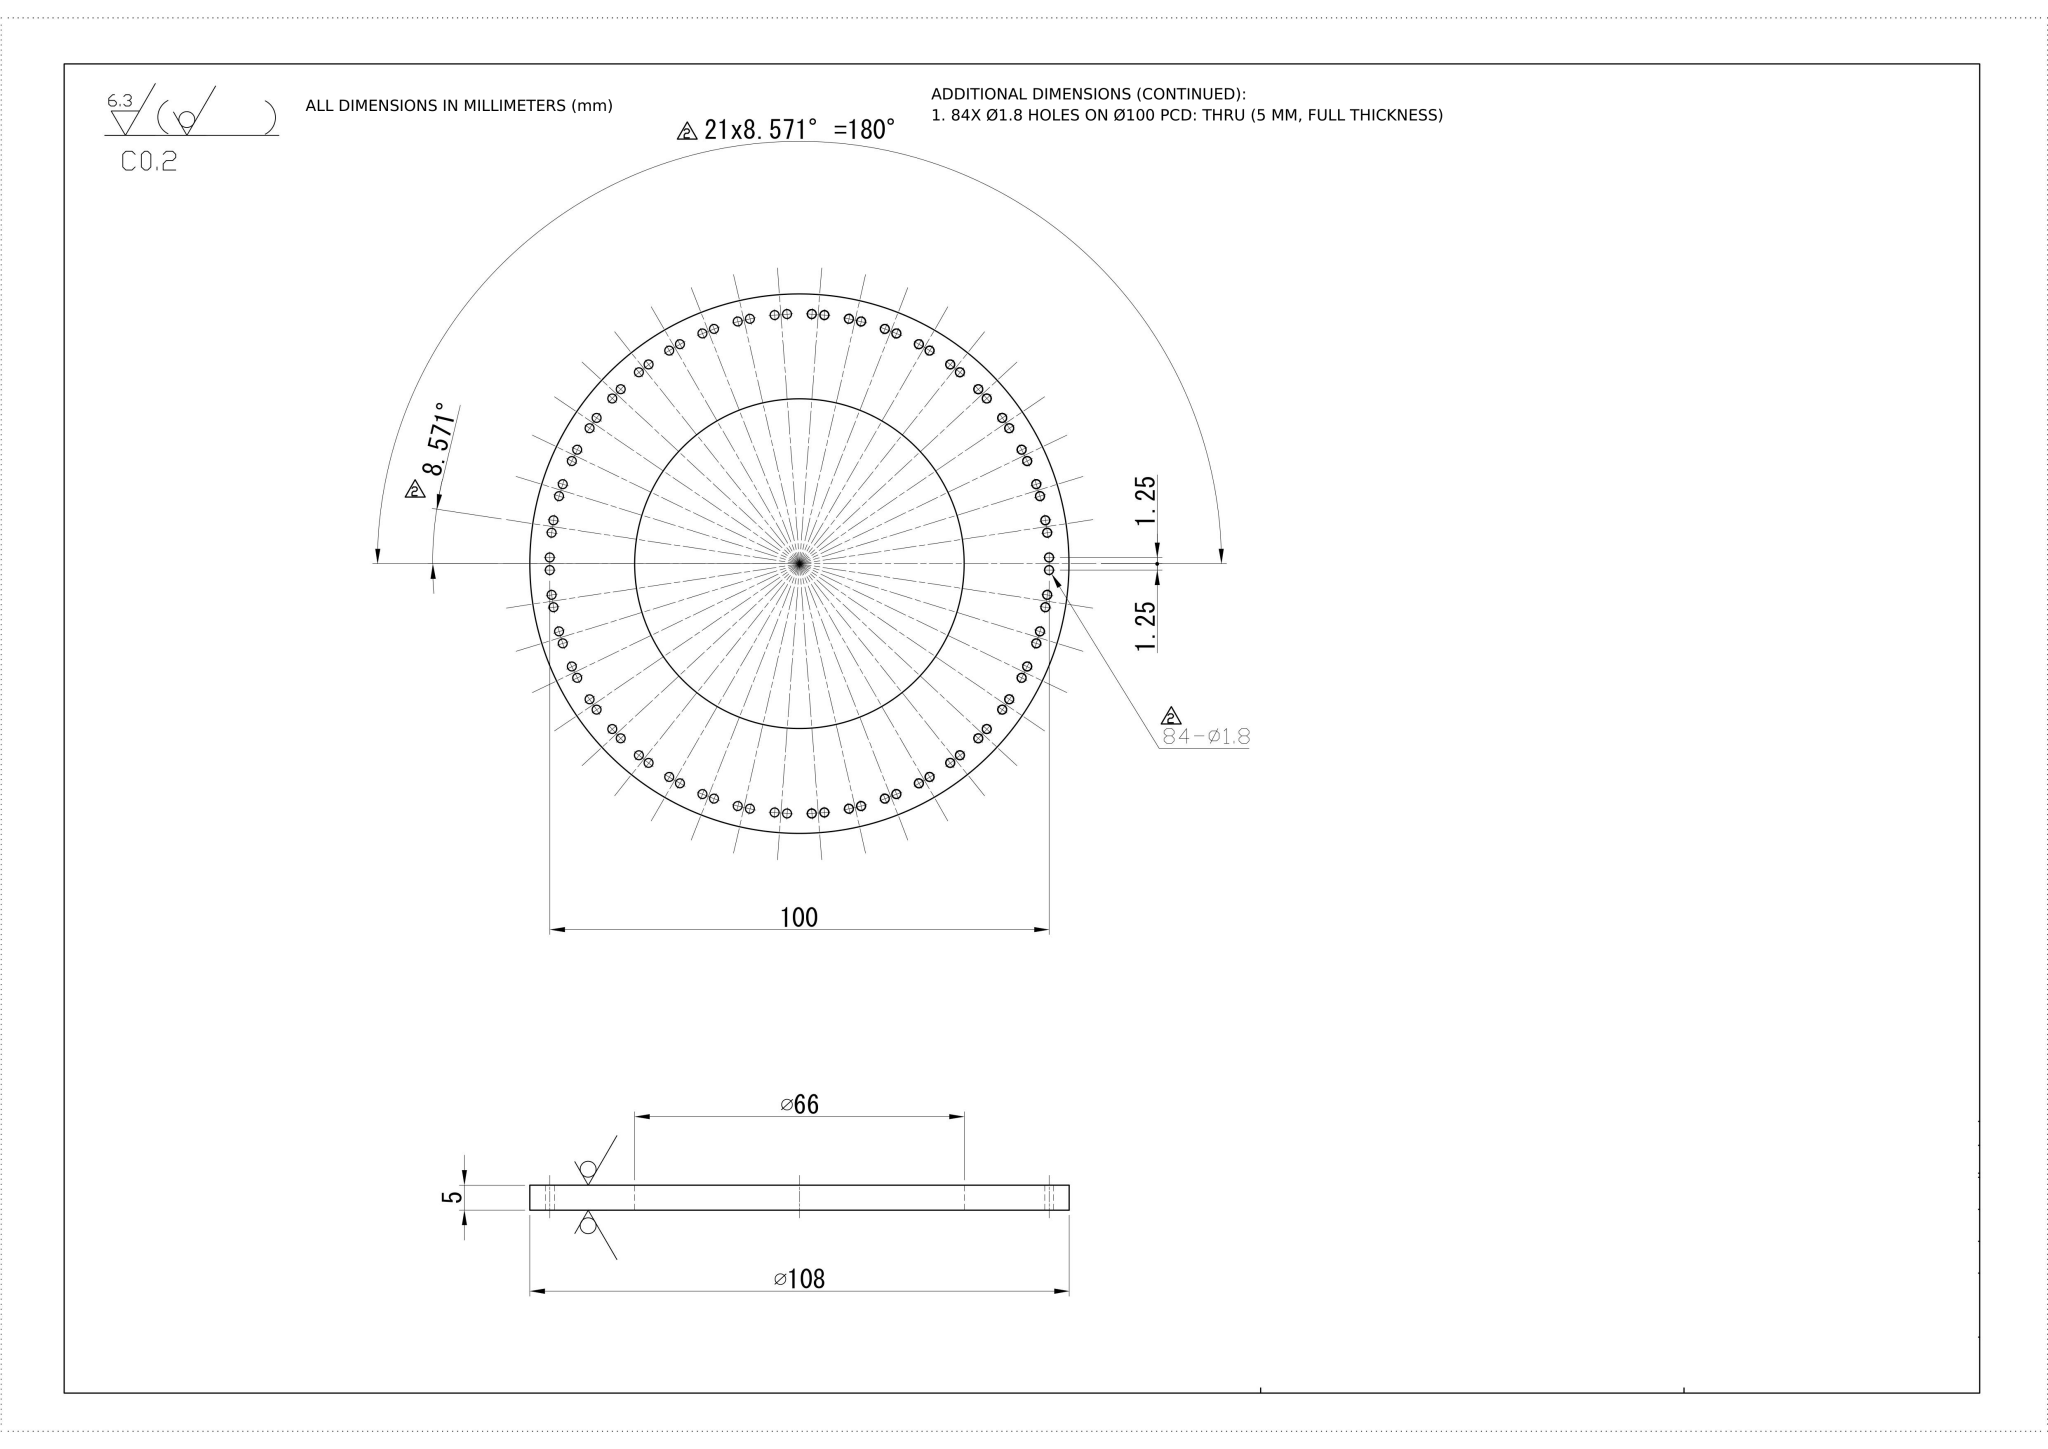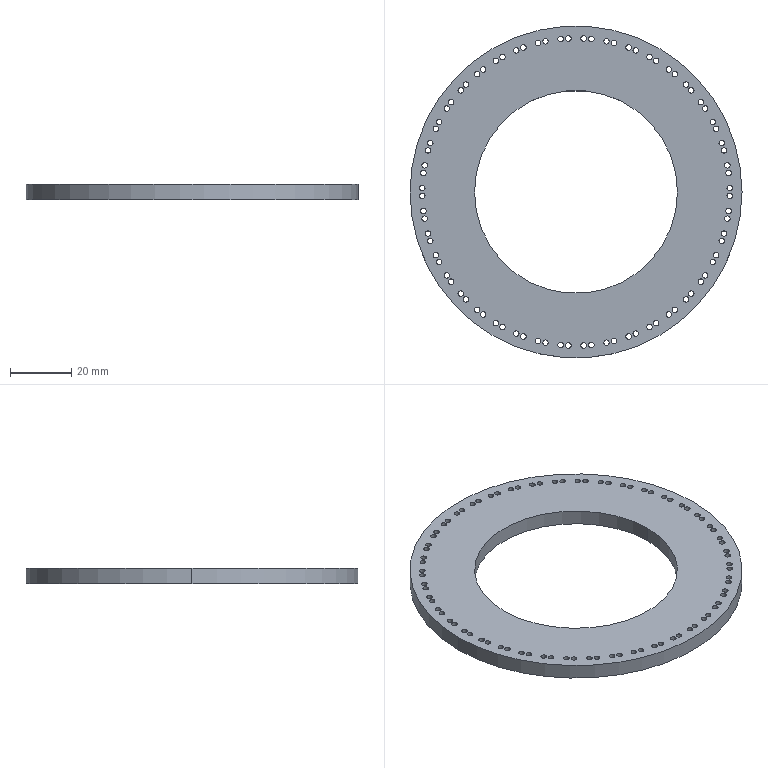Part | NX | mm | 1 solid | 174 faces | box 108 x 108 x 5 mm | volume 27630 mm3 | cylinder 172 | plane 2 | commonest cylinder face diameters 1.8 x168 66 x2 108 x2